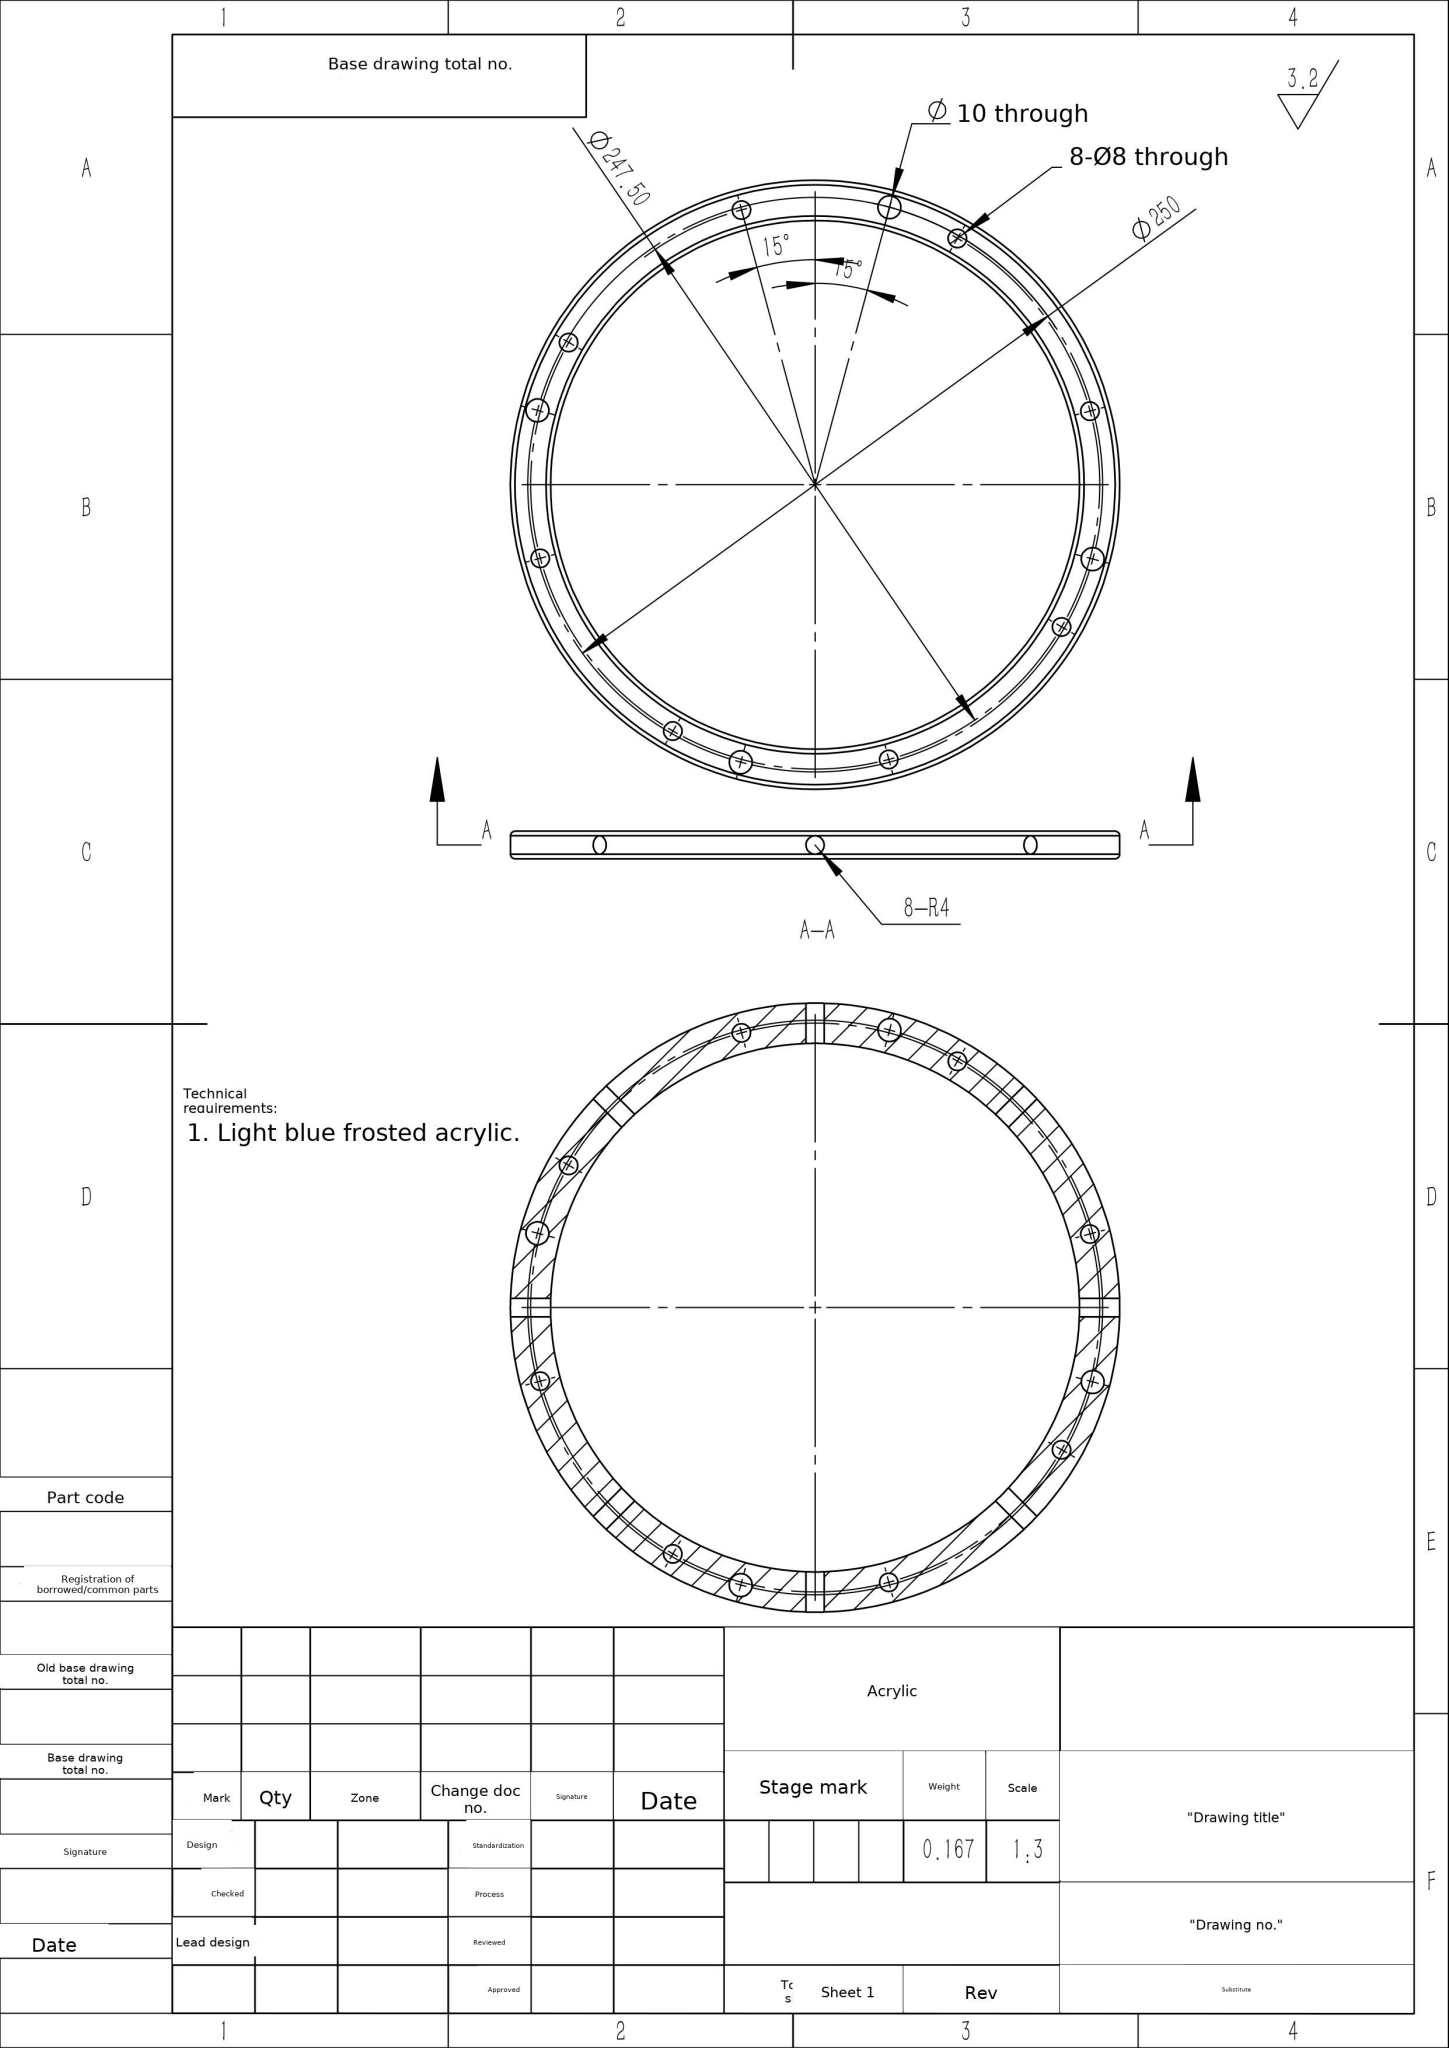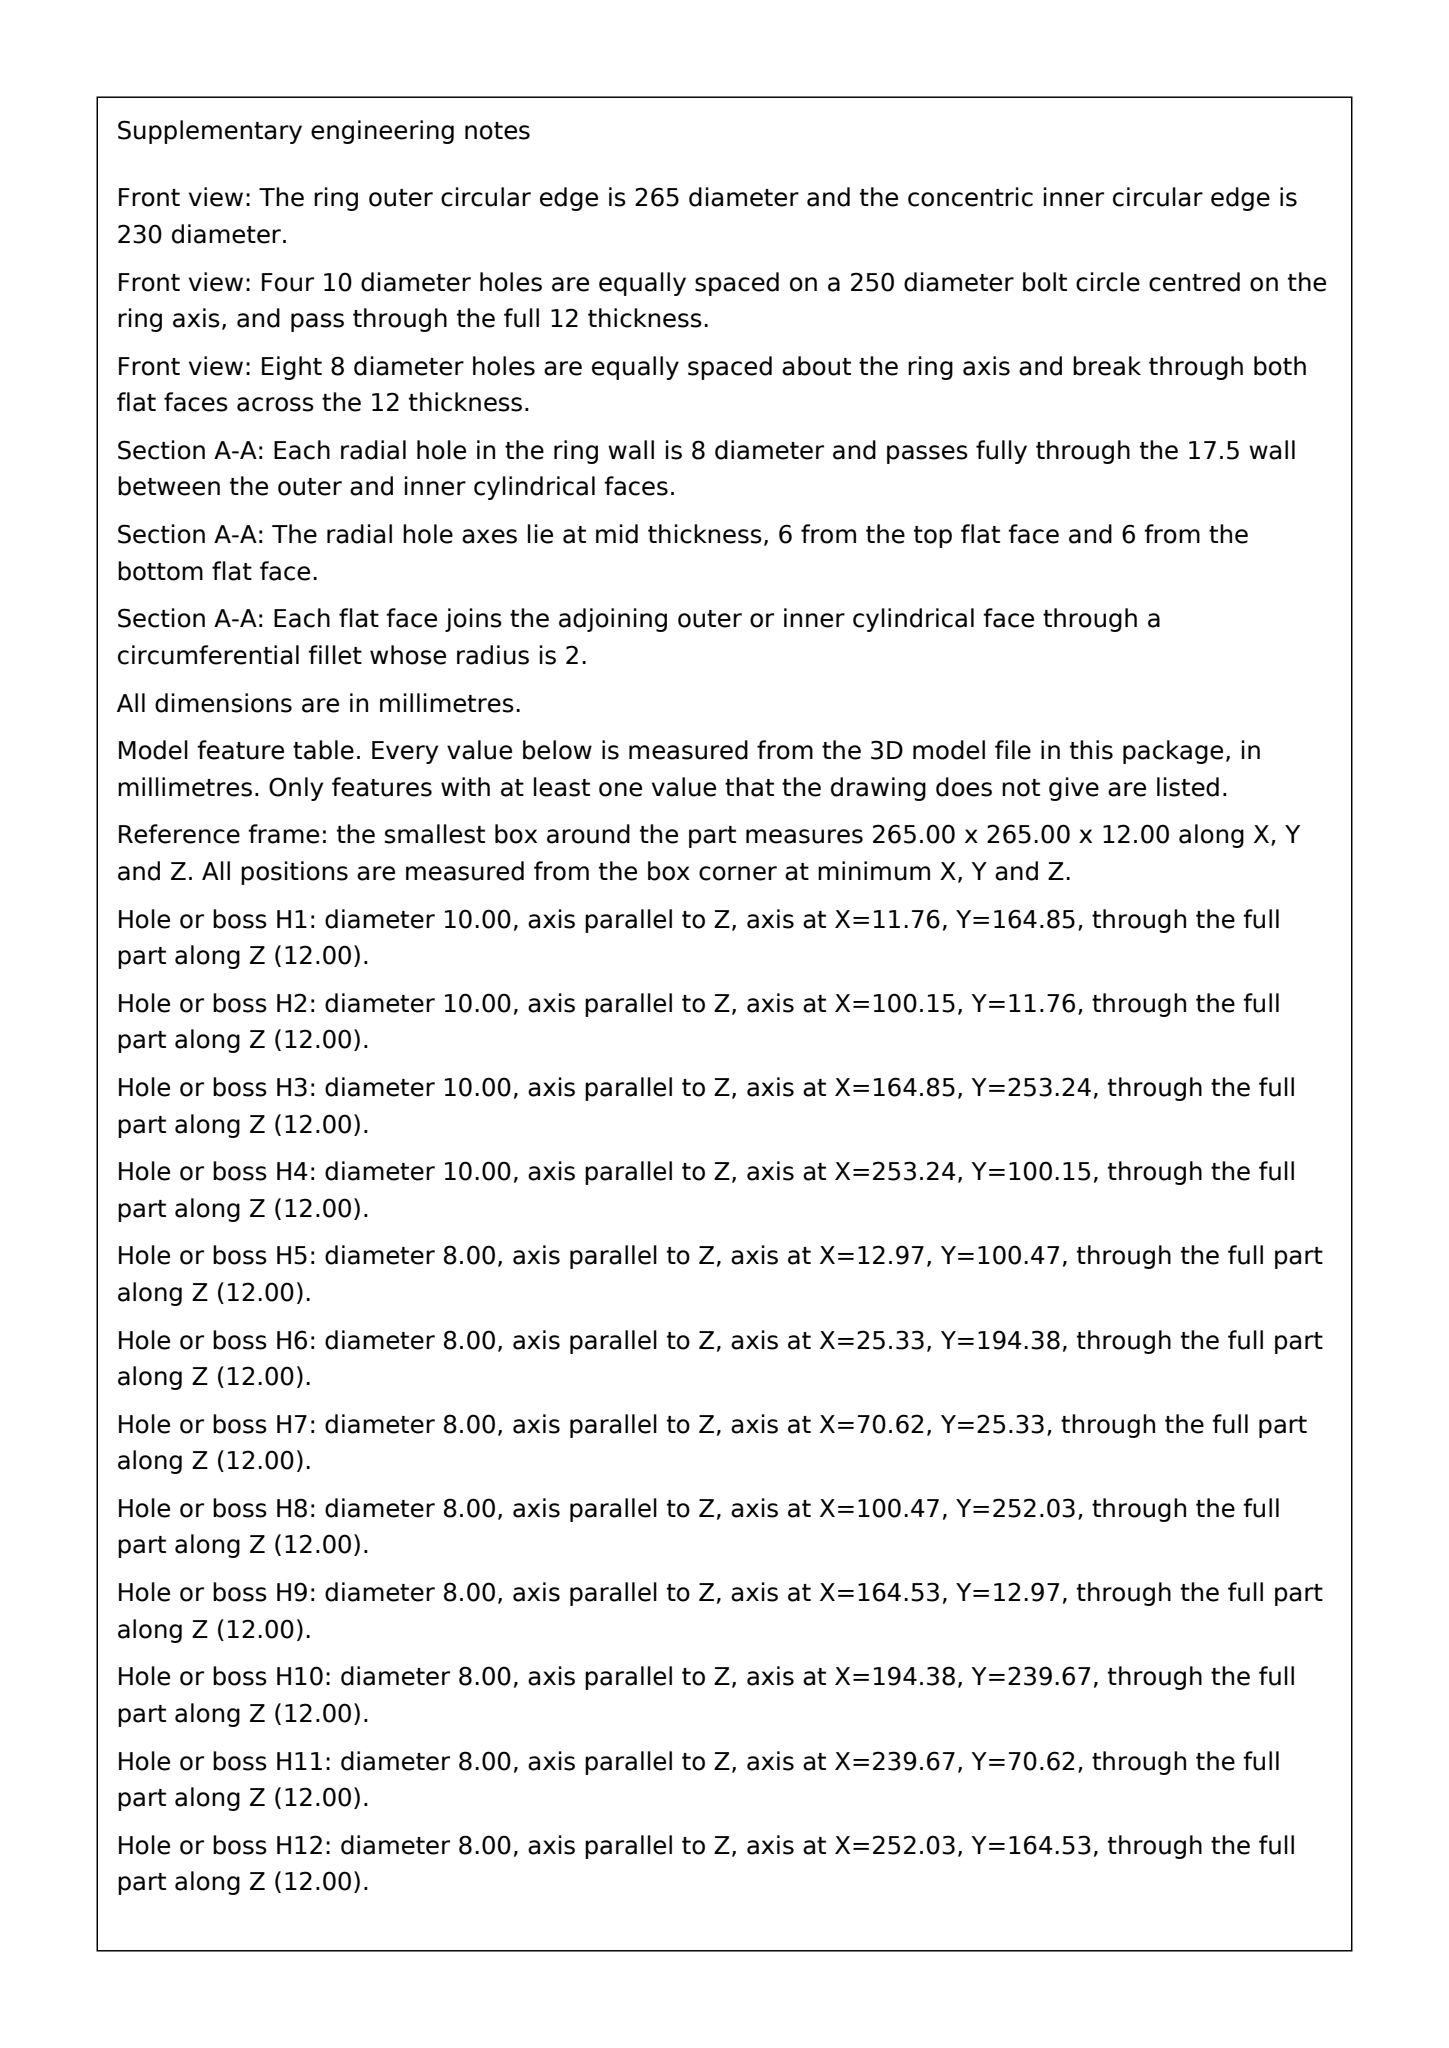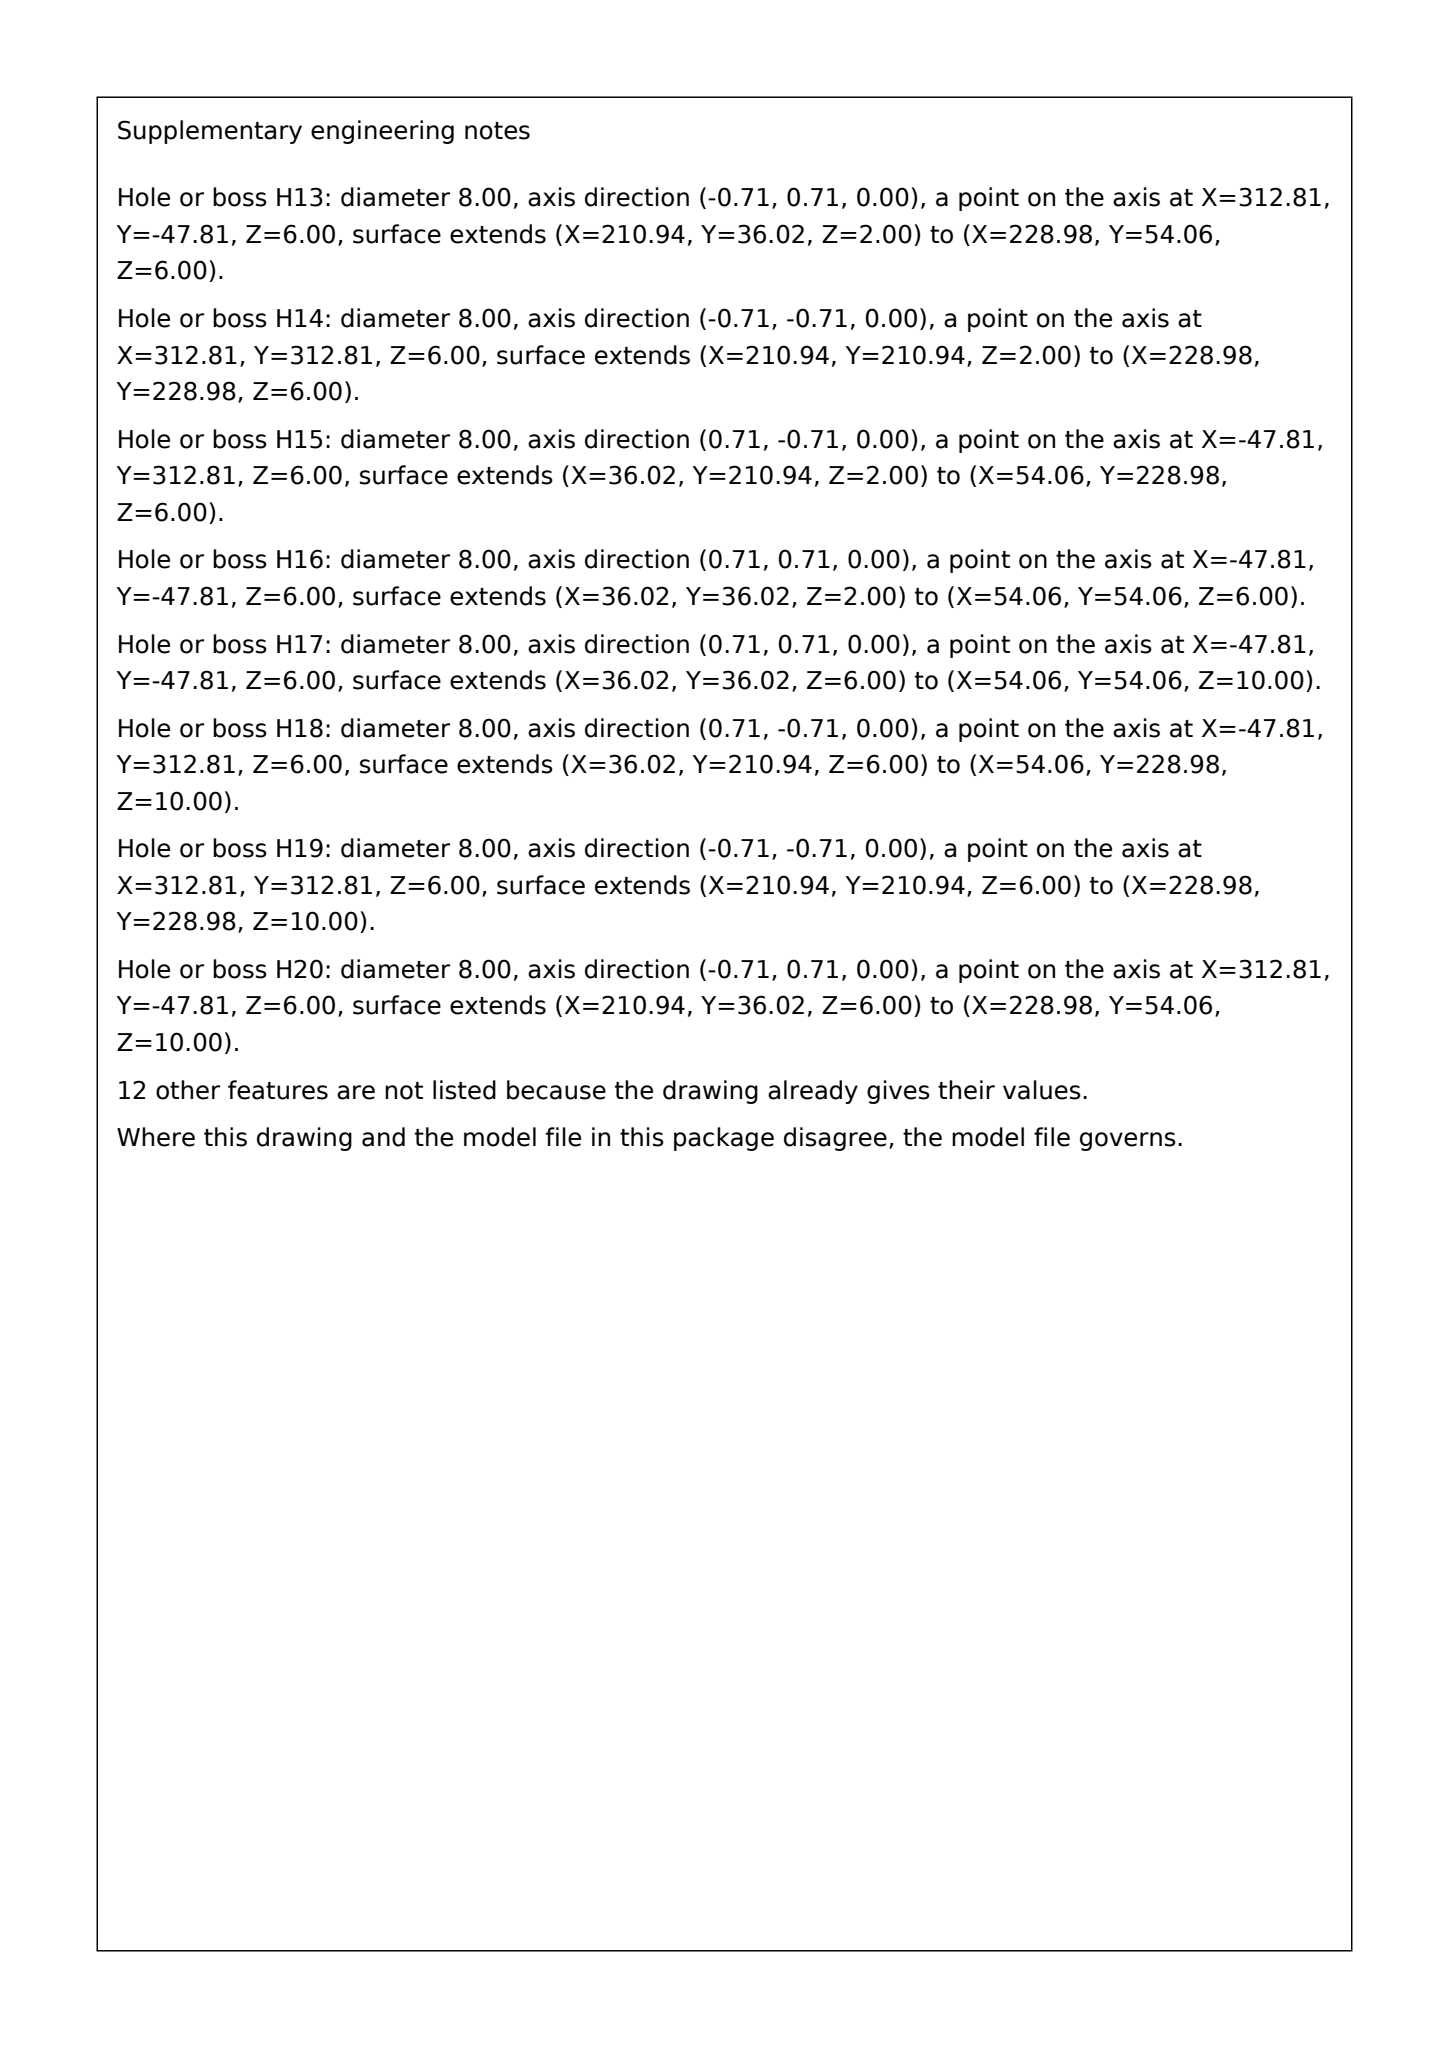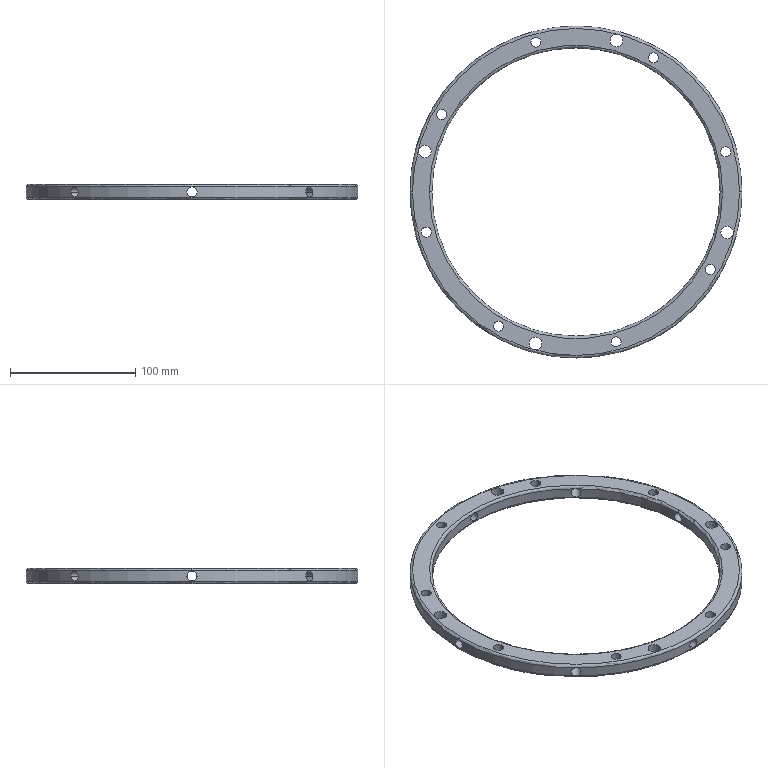Part | SolidWorks | mm | 1 solid | 66 faces | box 265 x 265 x 12 mm | volume 144981 mm3 | cylinder 56 | torus 8 | plane 2 | commonest cylinder face diameters 8 x32 10 x8 265 x8 230 x8
Drawing notes:
4-Ø10 THRU | from the solid: 4 cylinders dia 10.0, axis z, length 12.0 (full thk)
4-Ø10 EQ SP 90° ON Ø250 B.C., 15° FROM CL | from the solid: Ø10 holes at r=125.0 from ctr (143.42,143.42), angles 75/165/255/345°
8-R4 RADIAL HOLES EQ SP 45°, ON HORIZ/VERT CL | from the solid: 8 dia-8 radial cylinders: 2 axis x (y=143.42), 2 axis y (x=143.42), 4 on 45° lines thru ctr
8-R4 RADIAL HOLES ON MID-THK CL, 6 FROM EA FACE | from the solid: radial cyl axes at z=6.0; plates at z=0 and z=12.0
8-R4 = 8-Ø8 THRU WALL, Ø230 TO Ø265 | from the solid: radial cylinders dia 8.0, len 17.57 thru wall between Ø230 and Ø265
UNSPECIFIED FILLETS R2 (8 PLCS) | from the solid: fillet_radii [[2.0, 8]]
8-Ø8 THRU EQ SP 45° ON Ø247.50 B.C., 1ST HOLE 15° FROM HORIZ CL | from the solid: Eight Ø8 z-axis thru holes (L=12) at R=123.75 from center (143.42,143.42): angles 15°,60°,105°,150°,195°,240°,285°,330° = 45° equal spacing on Ø247.50 B.C.
build123d program:
from build123d import *

# Parameters (mm, degrees)
SKETCH1_R           = 132.5
SKETCH1_R_2         = 115
BOSS_EXTRUDE1_DEPTH = 6
FILLET1_R           = 2
SKETCH2_R           = 4
CUT_EXTRUDE1_DEPTH  = 255
CIRPATTERN1_COUNT   = 8
SKETCH3_R           = 5
CUT_EXTRUDE2_DEPTH  = 39
CIRPATTERN2_COUNT   = 4
SKETCH4_R           = 4
CUT_EXTRUDE3_DEPTH  = 39
CIRPATTERN3_COUNT   = 8


with BuildPart() as part:
    # Sketch1 → Boss-Extrude1 (new, symmetric)
    with BuildSketch(Plane.XY):
        Circle(SKETCH1_R)
        Circle(SKETCH1_R_2, mode=Mode.SUBTRACT)
    extrude(amount=BOSS_EXTRUDE1_DEPTH, both=True)

    # Fillet1
    fillet1_edges = [part.edges().sort_by_distance(p)[0] for p in [
        (-132.5, 0, -6),
        (-132.5, 0, 6),
        (-115, 0, -6),
        (-115, 0, 6),
    ]]
    fillet(fillet1_edges, radius=FILLET1_R)

    # Sketch2 → Cut-Extrude1 (cut)
    with BuildSketch(Plane(origin=(0, 0, 0), x_dir=(1, 0, 0), z_dir=(0, 1, 0))):
        with Locations(Location((0, 0, 0), (0, 0, 270))):
            Circle(SKETCH2_R)
    cut_extrude1 = extrude(amount=-CUT_EXTRUDE1_DEPTH, mode=Mode.SUBTRACT)

    # CirPattern1: Cut-Extrude1 ×8 about axis
    cirpattern1_axis = Axis((0, 0, 6), (0, 0, -1))
    for i in range(1, CIRPATTERN1_COUNT):
        add(cut_extrude1.rotate(cirpattern1_axis, i * 360 / CIRPATTERN1_COUNT), mode=Mode.SUBTRACT)

    # Sketch3 → Cut-Extrude2 (cut)
    with BuildSketch(Plane.XY.offset(6)):
        with Locations((32.352, 120.741)):
            Circle(SKETCH3_R)
    cut_extrude2 = extrude(amount=-CUT_EXTRUDE2_DEPTH, mode=Mode.SUBTRACT)

    # CirPattern2: Cut-Extrude2 ×4 about axis
    cirpattern2_axis = Axis((0, 0, 0), (0, 0, 1))
    for i in range(1, CIRPATTERN2_COUNT):
        add(cut_extrude2.rotate(cirpattern2_axis, i * 360 / CIRPATTERN2_COUNT), mode=Mode.SUBTRACT)

    # Sketch4 → Cut-Extrude3 (cut)
    with BuildSketch(Plane.XY.offset(6)):
        with Locations((61.875, 107.171)):
            Circle(SKETCH4_R)
    cut_extrude3 = extrude(amount=-CUT_EXTRUDE3_DEPTH, mode=Mode.SUBTRACT)

    # CirPattern3: Cut-Extrude3 ×8 about axis
    cirpattern3_axis = Axis((0, 0, 0), (0, 0, 1))
    for i in range(1, CIRPATTERN3_COUNT):
        add(cut_extrude3.rotate(cirpattern3_axis, i * 360 / CIRPATTERN3_COUNT), mode=Mode.SUBTRACT)


solid = part.part